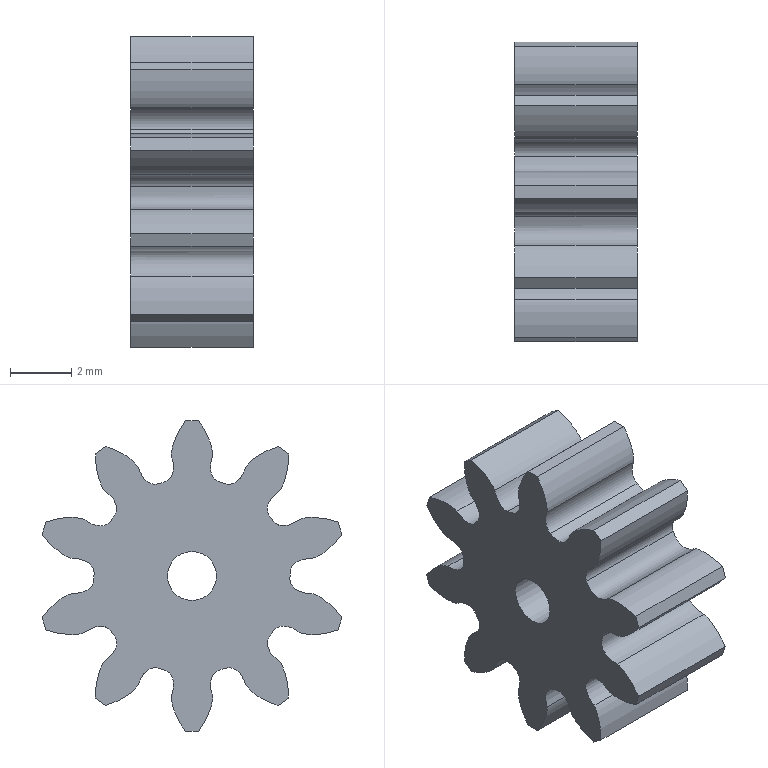Component | NX | GEAR_1_2 | 1 solid | 53 faces | volume 206 mm3 | spline 50 | plane 2 | cylinder 1 | commonest cylinder face diameters 1.6 x1